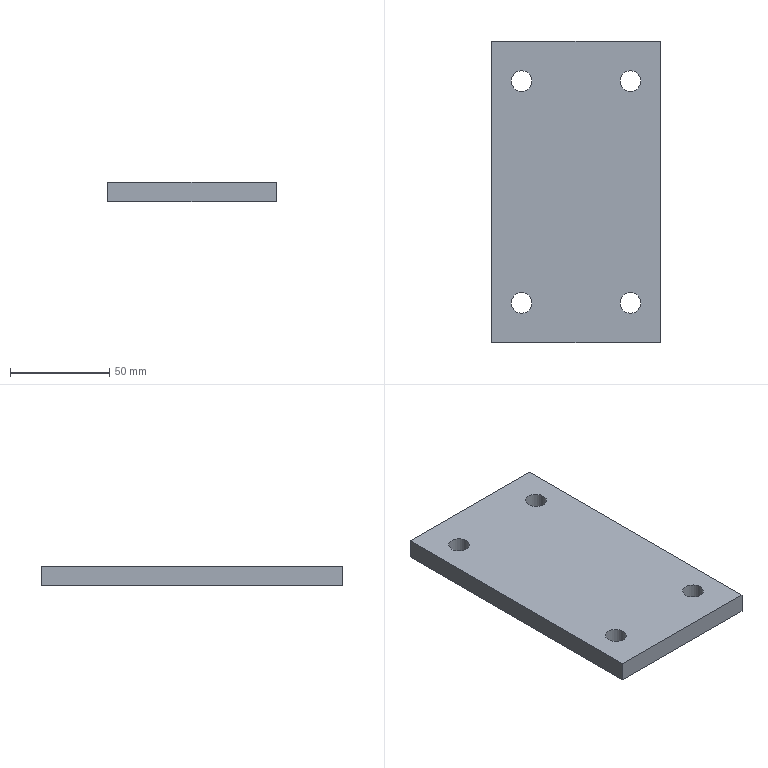Component | NX | FIXED_PLATE_7 | 1 solid | 10 faces | box 85 x 152 x 10 mm | volume 125736 mm3 | plane 6 | cylinder 4 | commonest cylinder face diameters 10.5 x4
STEP:
#1=CARTESIAN_POINT('',(0.,0.,0.));
#2=DIRECTION('',(0.,0.,1.));
#3=DIRECTION('',(1.,0.,0.));
#4=AXIS2_PLACEMENT_3D('',#1,#2,#3);
#5=CARTESIAN_POINT('',(1381.754,1330.,781.574));
#6=VERTEX_POINT('',#5);
#7=CARTESIAN_POINT('',(1381.754,1178.,781.574));
#8=VERTEX_POINT('',#7);
#9=CARTESIAN_POINT('',(1381.754,1330.,781.574));
#10=DIRECTION('',(0.,-1.,0.));
#11=VECTOR('',#10,1.);
#12=LINE('',#9,#11);
#13=CARTESIAN_POINT('',(1381.754,1330.,771.574));
#14=DIRECTION('',(-1.,0.,0.));
#15=DIRECTION('',(0.,0.,1.));
#16=AXIS2_PLACEMENT_3D('',#13,#14,#15);
#17=PLANE('',#16);
#18=CARTESIAN_POINT('',(10.,0.));
#19=DIRECTION('',(0.,-1.));
#20=VECTOR('',#19,1.);
#21=LINE('',#18,#20);
#22=(GEOMETRIC_REPRESENTATION_CONTEXT(2)PARAMETRIC_REPRESENTATION_CONTEXT()REPRESENTATION_CONTEXT('',''));
#23=DEFINITIONAL_REPRESENTATION('',(#21),#22);
#24=PCURVE('',#17,#23);
#25=CARTESIAN_POINT('',(1396.754,1198.,781.574));
#26=DIRECTION('',(0.,0.,1.));
#27=DIRECTION('',(1.,0.,0.));
#28=AXIS2_PLACEMENT_3D('',#25,#26,#27);
#29=PLANE('',#28);
#30=CARTESIAN_POINT('',(-15.,132.));
#31=DIRECTION('',(0.,-1.));
#32=VECTOR('',#31,1.);
#33=LINE('',#30,#32);
#34=(GEOMETRIC_REPRESENTATION_CONTEXT(2)PARAMETRIC_REPRESENTATION_CONTEXT()REPRESENTATION_CONTEXT('',''));
#35=DEFINITIONAL_REPRESENTATION('',(#33),#34);
#36=PCURVE('',#29,#35);
#37=SURFACE_CURVE('',#12,(#24,#36),.PCURVE_S1.);
#38=EDGE_CURVE('',#6,#8,#37,.T.);
#39=ORIENTED_EDGE('',*,*,#38,.F.);
#40=CARTESIAN_POINT('',(1381.754,1330.,771.574));
#41=VERTEX_POINT('',#40);
#42=CARTESIAN_POINT('',(1381.754,1330.,771.574));
#43=DIRECTION('',(0.,0.,1.));
#44=VECTOR('',#43,1.);
#45=LINE('',#42,#44);
#46=CARTESIAN_POINT('',(0.,0.));
#47=DIRECTION('',(1.,0.));
#48=VECTOR('',#47,1.);
#49=LINE('',#46,#48);
#50=(GEOMETRIC_REPRESENTATION_CONTEXT(2)PARAMETRIC_REPRESENTATION_CONTEXT()REPRESENTATION_CONTEXT('',''));
#51=DEFINITIONAL_REPRESENTATION('',(#49),#50);
#52=PCURVE('',#17,#51);
#53=CARTESIAN_POINT('',(1466.754,1330.,771.574));
#54=DIRECTION('',(0.,1.,0.));
#55=DIRECTION('',(0.,0.,1.));
#56=AXIS2_PLACEMENT_3D('',#53,#54,#55);
#57=PLANE('',#56);
#58=CARTESIAN_POINT('',(0.,-85.));
#59=DIRECTION('',(1.,0.));
#60=VECTOR('',#59,1.);
#61=LINE('',#58,#60);
#62=(GEOMETRIC_REPRESENTATION_CONTEXT(2)PARAMETRIC_REPRESENTATION_CONTEXT()REPRESENTATION_CONTEXT('',''));
#63=DEFINITIONAL_REPRESENTATION('',(#61),#62);
#64=PCURVE('',#57,#63);
#65=SURFACE_CURVE('',#45,(#52,#64),.PCURVE_S1.);
#66=EDGE_CURVE('',#41,#6,#65,.T.);
#67=ORIENTED_EDGE('',*,*,#66,.F.);
#68=CARTESIAN_POINT('',(1381.754,1178.,771.574));
#69=VERTEX_POINT('',#68);
#70=CARTESIAN_POINT('',(1381.754,1330.,771.574));
#71=DIRECTION('',(0.,-1.,0.));
#72=VECTOR('',#71,1.);
#73=LINE('',#70,#72);
#74=CARTESIAN_POINT('',(0.,0.));
#75=DIRECTION('',(0.,-1.));
#76=VECTOR('',#75,1.);
#77=LINE('',#74,#76);
#78=(GEOMETRIC_REPRESENTATION_CONTEXT(2)PARAMETRIC_REPRESENTATION_CONTEXT()REPRESENTATION_CONTEXT('',''));
#79=DEFINITIONAL_REPRESENTATION('',(#77),#78);
#80=PCURVE('',#17,#79);
#81=CARTESIAN_POINT('',(1396.754,1198.,771.574));
#82=DIRECTION('',(0.,0.,1.));
#83=DIRECTION('',(1.,0.,0.));
#84=AXIS2_PLACEMENT_3D('',#81,#82,#83);
#85=PLANE('',#84);
#86=CARTESIAN_POINT('',(-15.,132.));
#87=DIRECTION('',(0.,-1.));
#88=VECTOR('',#87,1.);
#89=LINE('',#86,#88);
#90=(GEOMETRIC_REPRESENTATION_CONTEXT(2)PARAMETRIC_REPRESENTATION_CONTEXT()REPRESENTATION_CONTEXT('',''));
#91=DEFINITIONAL_REPRESENTATION('',(#89),#90);
#92=PCURVE('',#85,#91);
#93=SURFACE_CURVE('',#73,(#80,#92),.PCURVE_S1.);
#94=EDGE_CURVE('',#41,#69,#93,.T.);
#95=ORIENTED_EDGE('',*,*,#94,.T.);
#96=CARTESIAN_POINT('',(1381.754,1178.,771.574));
#97=DIRECTION('',(0.,0.,1.));
#98=VECTOR('',#97,1.);
#99=LINE('',#96,#98);
#100=CARTESIAN_POINT('',(0.,-152.));
#101=DIRECTION('',(1.,0.));
#102=VECTOR('',#101,1.);
#103=LINE('',#100,#102);
#104=(GEOMETRIC_REPRESENTATION_CONTEXT(2)PARAMETRIC_REPRESENTATION_CONTEXT()REPRESENTATION_CONTEXT('',''));
#105=DEFINITIONAL_REPRESENTATION('',(#103),#104);
#106=PCURVE('',#17,#105);
#107=CARTESIAN_POINT('',(1381.754,1178.,771.574));
#108=DIRECTION('',(0.,-1.,0.));
#109=DIRECTION('',(0.,0.,-1.));
#110=AXIS2_PLACEMENT_3D('',#107,#108,#109);
#111=PLANE('',#110);
#112=CARTESIAN_POINT('',(0.,0.));
#113=DIRECTION('',(-1.,0.));
#114=VECTOR('',#113,1.);
#115=LINE('',#112,#114);
#116=(GEOMETRIC_REPRESENTATION_CONTEXT(2)PARAMETRIC_REPRESENTATION_CONTEXT()REPRESENTATION_CONTEXT('',''));
#117=DEFINITIONAL_REPRESENTATION('',(#115),#116);
#118=PCURVE('',#111,#117);
#119=SURFACE_CURVE('',#99,(#106,#118),.PCURVE_S1.);
#120=EDGE_CURVE('',#69,#8,#119,.T.);
#121=ORIENTED_EDGE('',*,*,#120,.T.);
#122=EDGE_LOOP('',(#39,#67,#95,#121));
#123=FACE_BOUND('',#122,.T.);
#124=ADVANCED_FACE('',(#123),#17,.T.);
#125=CARTESIAN_POINT('',(1466.754,1178.,781.574));
#126=VERTEX_POINT('',#125);
#127=CARTESIAN_POINT('',(1381.754,1178.,781.574));
#128=DIRECTION('',(1.,0.,0.));
#129=VECTOR('',#128,1.);
#130=LINE('',#127,#129);
#131=CARTESIAN_POINT('',(-10.,0.));
#132=DIRECTION('',(0.,1.));
#133=VECTOR('',#132,1.);
#134=LINE('',#131,#133);
#135=(GEOMETRIC_REPRESENTATION_CONTEXT(2)PARAMETRIC_REPRESENTATION_CONTEXT()REPRESENTATION_CONTEXT('',''));
#136=DEFINITIONAL_REPRESENTATION('',(#134),#135);
#137=PCURVE('',#111,#136);
#138=CARTESIAN_POINT('',(-15.,-20.));
#139=DIRECTION('',(1.,0.));
#140=VECTOR('',#139,1.);
#141=LINE('',#138,#140);
#142=(GEOMETRIC_REPRESENTATION_CONTEXT(2)PARAMETRIC_REPRESENTATION_CONTEXT()REPRESENTATION_CONTEXT('',''));
#143=DEFINITIONAL_REPRESENTATION('',(#141),#142);
#144=PCURVE('',#29,#143);
#145=SURFACE_CURVE('',#130,(#137,#144),.PCURVE_S1.);
#146=EDGE_CURVE('',#8,#126,#145,.T.);
#147=ORIENTED_EDGE('',*,*,#146,.F.);
#148=ORIENTED_EDGE('',*,*,#120,.F.);
#149=CARTESIAN_POINT('',(1466.754,1178.,771.574));
#150=VERTEX_POINT('',#149);
#151=CARTESIAN_POINT('',(1381.754,1178.,771.574));
#152=DIRECTION('',(1.,0.,0.));
#153=VECTOR('',#152,1.);
#154=LINE('',#151,#153);
#155=CARTESIAN_POINT('',(0.,0.));
#156=DIRECTION('',(0.,1.));
#157=VECTOR('',#156,1.);
#158=LINE('',#155,#157);
#159=(GEOMETRIC_REPRESENTATION_CONTEXT(2)PARAMETRIC_REPRESENTATION_CONTEXT()REPRESENTATION_CONTEXT('',''));
#160=DEFINITIONAL_REPRESENTATION('',(#158),#159);
#161=PCURVE('',#111,#160);
#162=CARTESIAN_POINT('',(-15.,-20.));
#163=DIRECTION('',(1.,0.));
#164=VECTOR('',#163,1.);
#165=LINE('',#162,#164);
#166=(GEOMETRIC_REPRESENTATION_CONTEXT(2)PARAMETRIC_REPRESENTATION_CONTEXT()REPRESENTATION_CONTEXT('',''));
#167=DEFINITIONAL_REPRESENTATION('',(#165),#166);
#168=PCURVE('',#85,#167);
#169=SURFACE_CURVE('',#154,(#161,#168),.PCURVE_S1.);
#170=EDGE_CURVE('',#69,#150,#169,.T.);
#171=ORIENTED_EDGE('',*,*,#170,.T.);
#172=CARTESIAN_POINT('',(1466.754,1178.,771.574));
#173=DIRECTION('',(0.,0.,1.));
#174=VECTOR('',#173,1.);
#175=LINE('',#172,#174);
#176=CARTESIAN_POINT('',(0.,85.));
#177=DIRECTION('',(-1.,0.));
#178=VECTOR('',#177,1.);
#179=LINE('',#176,#178);
#180=(GEOMETRIC_REPRESENTATION_CONTEXT(2)PARAMETRIC_REPRESENTATION_CONTEXT()REPRESENTATION_CONTEXT('',''));
#181=DEFINITIONAL_REPRESENTATION('',(#179),#180);
#182=PCURVE('',#111,#181);
#183=CARTESIAN_POINT('',(1466.754,1178.,771.574));
#184=DIRECTION('',(1.,-0.,0.));
#185=DIRECTION('',(0.,1.,0.));
#186=AXIS2_PLACEMENT_3D('',#183,#184,#185);
#187=PLANE('',#186);
#188=CARTESIAN_POINT('',(0.,0.));
#189=DIRECTION('',(0.,1.));
#190=VECTOR('',#189,1.);
#191=LINE('',#188,#190);
#192=(GEOMETRIC_REPRESENTATION_CONTEXT(2)PARAMETRIC_REPRESENTATION_CONTEXT()REPRESENTATION_CONTEXT('',''));
#193=DEFINITIONAL_REPRESENTATION('',(#191),#192);
#194=PCURVE('',#187,#193);
#195=SURFACE_CURVE('',#175,(#182,#194),.PCURVE_S1.);
#196=EDGE_CURVE('',#150,#126,#195,.T.);
#197=ORIENTED_EDGE('',*,*,#196,.T.);
#198=EDGE_LOOP('',(#147,#148,#171,#197));
#199=FACE_BOUND('',#198,.T.);
#200=ADVANCED_FACE('',(#199),#111,.T.);
#201=CARTESIAN_POINT('',(1466.754,1330.,781.574));
#202=VERTEX_POINT('',#201);
#203=CARTESIAN_POINT('',(1466.754,1178.,781.574));
#204=DIRECTION('',(0.,1.,0.));
#205=VECTOR('',#204,1.);
#206=LINE('',#203,#205);
#207=CARTESIAN_POINT('',(0.,10.));
#208=DIRECTION('',(1.,0.));
#209=VECTOR('',#208,1.);
#210=LINE('',#207,#209);
#211=(GEOMETRIC_REPRESENTATION_CONTEXT(2)PARAMETRIC_REPRESENTATION_CONTEXT()REPRESENTATION_CONTEXT('',''));
#212=DEFINITIONAL_REPRESENTATION('',(#210),#211);
#213=PCURVE('',#187,#212);
#214=CARTESIAN_POINT('',(70.,-20.));
#215=DIRECTION('',(0.,1.));
#216=VECTOR('',#215,1.);
#217=LINE('',#214,#216);
#218=(GEOMETRIC_REPRESENTATION_CONTEXT(2)PARAMETRIC_REPRESENTATION_CONTEXT()REPRESENTATION_CONTEXT('',''));
#219=DEFINITIONAL_REPRESENTATION('',(#217),#218);
#220=PCURVE('',#29,#219);
#221=SURFACE_CURVE('',#206,(#213,#220),.PCURVE_S1.);
#222=EDGE_CURVE('',#126,#202,#221,.T.);
#223=ORIENTED_EDGE('',*,*,#222,.F.);
#224=ORIENTED_EDGE('',*,*,#196,.F.);
#225=CARTESIAN_POINT('',(1466.754,1330.,771.574));
#226=VERTEX_POINT('',#225);
#227=CARTESIAN_POINT('',(1466.754,1178.,771.574));
#228=DIRECTION('',(0.,1.,0.));
#229=VECTOR('',#228,1.);
#230=LINE('',#227,#229);
#231=CARTESIAN_POINT('',(0.,0.));
#232=DIRECTION('',(1.,0.));
#233=VECTOR('',#232,1.);
#234=LINE('',#231,#233);
#235=(GEOMETRIC_REPRESENTATION_CONTEXT(2)PARAMETRIC_REPRESENTATION_CONTEXT()REPRESENTATION_CONTEXT('',''));
#236=DEFINITIONAL_REPRESENTATION('',(#234),#235);
#237=PCURVE('',#187,#236);
#238=CARTESIAN_POINT('',(70.,-20.));
#239=DIRECTION('',(0.,1.));
#240=VECTOR('',#239,1.);
#241=LINE('',#238,#240);
#242=(GEOMETRIC_REPRESENTATION_CONTEXT(2)PARAMETRIC_REPRESENTATION_CONTEXT()REPRESENTATION_CONTEXT('',''));
#243=DEFINITIONAL_REPRESENTATION('',(#241),#242);
#244=PCURVE('',#85,#243);
#245=SURFACE_CURVE('',#230,(#237,#244),.PCURVE_S1.);
#246=EDGE_CURVE('',#150,#226,#245,.T.);
#247=ORIENTED_EDGE('',*,*,#246,.T.);
#248=CARTESIAN_POINT('',(1466.754,1330.,771.574));
#249=DIRECTION('',(0.,0.,1.));
#250=VECTOR('',#249,1.);
#251=LINE('',#248,#250);
#252=CARTESIAN_POINT('',(152.,0.));
#253=DIRECTION('',(0.,1.));
#254=VECTOR('',#253,1.);
#255=LINE('',#252,#254);
#256=(GEOMETRIC_REPRESENTATION_CONTEXT(2)PARAMETRIC_REPRESENTATION_CONTEXT()REPRESENTATION_CONTEXT('',''));
#257=DEFINITIONAL_REPRESENTATION('',(#255),#256);
#258=PCURVE('',#187,#257);
#259=CARTESIAN_POINT('',(0.,0.));
#260=DIRECTION('',(1.,0.));
#261=VECTOR('',#260,1.);
#262=LINE('',#259,#261);
#263=(GEOMETRIC_REPRESENTATION_CONTEXT(2)PARAMETRIC_REPRESENTATION_CONTEXT()REPRESENTATION_CONTEXT('',''));
#264=DEFINITIONAL_REPRESENTATION('',(#262),#263);
#265=PCURVE('',#57,#264);
#266=SURFACE_CURVE('',#251,(#258,#265),.PCURVE_S1.);
#267=EDGE_CURVE('',#226,#202,#266,.T.);
#268=ORIENTED_EDGE('',*,*,#267,.T.);
#269=EDGE_LOOP('',(#223,#224,#247,#268));
#270=FACE_BOUND('',#269,.T.);
#271=ADVANCED_FACE('',(#270),#187,.T.);
#272=CARTESIAN_POINT('',(1457.004,1198.,771.574));
#273=VERTEX_POINT('',#272);
#274=CARTESIAN_POINT('',(1451.754,1198.,771.574));
#275=DIRECTION('',(0.,0.,1.));
#276=DIRECTION('',(1.,0.,0.));
#277=AXIS2_PLACEMENT_3D('',#274,#275,#276);
#278=CIRCLE('',#277,5.25);
#279=CARTESIAN_POINT('',(1451.754,1198.,771.574));
#280=DIRECTION('',(0.,0.,1.));
#281=DIRECTION('',(1.,0.,0.));
#282=AXIS2_PLACEMENT_3D('',#279,#280,#281);
#283=CYLINDRICAL_SURFACE('',#282,5.25);
#284=CARTESIAN_POINT('',(0.,0.));
#285=DIRECTION('',(1.,0.));
#286=VECTOR('',#285,1.);
#287=LINE('',#284,#286);
#288=(GEOMETRIC_REPRESENTATION_CONTEXT(2)PARAMETRIC_REPRESENTATION_CONTEXT()REPRESENTATION_CONTEXT('',''));
#289=DEFINITIONAL_REPRESENTATION('',(#287),#288);
#290=PCURVE('',#283,#289);
#291=CARTESIAN_POINT('',(55.,0.));
#292=DIRECTION('',(1.,0.));
#293=AXIS2_PLACEMENT_2D('',#291,#292);
#294=CIRCLE('',#293,5.25);
#295=(GEOMETRIC_REPRESENTATION_CONTEXT(2)PARAMETRIC_REPRESENTATION_CONTEXT()REPRESENTATION_CONTEXT('',''));
#296=DEFINITIONAL_REPRESENTATION('',(#294),#295);
#297=PCURVE('',#85,#296);
#298=SURFACE_CURVE('',#278,(#290,#297),.PCURVE_S1.);
#299=EDGE_CURVE('',#273,#273,#298,.T.);
#300=ORIENTED_EDGE('',*,*,#299,.T.);
#301=CARTESIAN_POINT('',(1457.004,1198.,781.574));
#302=VERTEX_POINT('',#301);
#303=CARTESIAN_POINT('',(1457.004,1198.,771.574));
#304=CARTESIAN_POINT('',(1457.004,1198.,781.574));
#305=B_SPLINE_CURVE_WITH_KNOTS('',1,(#303,#304),.UNSPECIFIED.,.F.,.F.,(2,2),(0.,10.),.PIECEWISE_BEZIER_KNOTS.);
#306=CARTESIAN_POINT('',(6.283,0.));
#307=DIRECTION('',(0.,1.));
#308=VECTOR('',#307,1.);
#309=LINE('',#306,#308);
#310=(GEOMETRIC_REPRESENTATION_CONTEXT(2)PARAMETRIC_REPRESENTATION_CONTEXT()REPRESENTATION_CONTEXT('',''));
#311=DEFINITIONAL_REPRESENTATION('',(#309),#310);
#312=PCURVE('',#283,#311);
#313=CARTESIAN_POINT('',(0.,0.));
#314=DIRECTION('',(0.,1.));
#315=VECTOR('',#314,1.);
#316=LINE('',#313,#315);
#317=(GEOMETRIC_REPRESENTATION_CONTEXT(2)PARAMETRIC_REPRESENTATION_CONTEXT()REPRESENTATION_CONTEXT('',''));
#318=DEFINITIONAL_REPRESENTATION('',(#316),#317);
#319=PCURVE('',#283,#318);
#320=SEAM_CURVE('',#305,(#312,#319),.PCURVE_S1.);
#321=EDGE_CURVE('',#273,#302,#320,.T.);
#322=ORIENTED_EDGE('',*,*,#321,.T.);
#323=CARTESIAN_POINT('',(1451.754,1198.,781.574));
#324=DIRECTION('',(0.,0.,1.));
#325=DIRECTION('',(1.,0.,0.));
#326=AXIS2_PLACEMENT_3D('',#323,#324,#325);
#327=CIRCLE('',#326,5.25);
#328=CARTESIAN_POINT('',(0.,10.));
#329=DIRECTION('',(1.,0.));
#330=VECTOR('',#329,1.);
#331=LINE('',#328,#330);
#332=(GEOMETRIC_REPRESENTATION_CONTEXT(2)PARAMETRIC_REPRESENTATION_CONTEXT()REPRESENTATION_CONTEXT('',''));
#333=DEFINITIONAL_REPRESENTATION('',(#331),#332);
#334=PCURVE('',#283,#333);
#335=CARTESIAN_POINT('',(55.,0.));
#336=DIRECTION('',(1.,0.));
#337=AXIS2_PLACEMENT_2D('',#335,#336);
#338=CIRCLE('',#337,5.25);
#339=(GEOMETRIC_REPRESENTATION_CONTEXT(2)PARAMETRIC_REPRESENTATION_CONTEXT()REPRESENTATION_CONTEXT('',''));
#340=DEFINITIONAL_REPRESENTATION('',(#338),#339);
#341=PCURVE('',#29,#340);
#342=SURFACE_CURVE('',#327,(#334,#341),.PCURVE_S1.);
#343=EDGE_CURVE('',#302,#302,#342,.T.);
#344=ORIENTED_EDGE('',*,*,#343,.F.);
#345=ORIENTED_EDGE('',*,*,#321,.F.);
#346=EDGE_LOOP('',(#300,#322,#344,#345));
#347=FACE_BOUND('',#346,.F.);
#348=ADVANCED_FACE('',(#347),#283,.F.);
#349=CARTESIAN_POINT('',(1402.004,1310.,771.574));
#350=VERTEX_POINT('',#349);
#351=CARTESIAN_POINT('',(1396.754,1310.,771.574));
#352=DIRECTION('',(0.,0.,1.));
#353=DIRECTION('',(1.,0.,0.));
#354=AXIS2_PLACEMENT_3D('',#351,#352,#353);
#355=CIRCLE('',#354,5.25);
#356=CARTESIAN_POINT('',(1396.754,1310.,771.574));
#357=DIRECTION('',(0.,0.,1.));
#358=DIRECTION('',(1.,0.,0.));
#359=AXIS2_PLACEMENT_3D('',#356,#357,#358);
#360=CYLINDRICAL_SURFACE('',#359,5.25);
#361=CARTESIAN_POINT('',(0.,0.));
#362=DIRECTION('',(1.,0.));
#363=VECTOR('',#362,1.);
#364=LINE('',#361,#363);
#365=(GEOMETRIC_REPRESENTATION_CONTEXT(2)PARAMETRIC_REPRESENTATION_CONTEXT()REPRESENTATION_CONTEXT('',''));
#366=DEFINITIONAL_REPRESENTATION('',(#364),#365);
#367=PCURVE('',#360,#366);
#368=CARTESIAN_POINT('',(0.,112.));
#369=DIRECTION('',(1.,0.));
#370=AXIS2_PLACEMENT_2D('',#368,#369);
#371=CIRCLE('',#370,5.25);
#372=(GEOMETRIC_REPRESENTATION_CONTEXT(2)PARAMETRIC_REPRESENTATION_CONTEXT()REPRESENTATION_CONTEXT('',''));
#373=DEFINITIONAL_REPRESENTATION('',(#371),#372);
#374=PCURVE('',#85,#373);
#375=SURFACE_CURVE('',#355,(#367,#374),.PCURVE_S1.);
#376=EDGE_CURVE('',#350,#350,#375,.T.);
#377=ORIENTED_EDGE('',*,*,#376,.T.);
#378=CARTESIAN_POINT('',(1402.004,1310.,781.574));
#379=VERTEX_POINT('',#378);
#380=CARTESIAN_POINT('',(1402.004,1310.,771.574));
#381=CARTESIAN_POINT('',(1402.004,1310.,781.574));
#382=B_SPLINE_CURVE_WITH_KNOTS('',1,(#380,#381),.UNSPECIFIED.,.F.,.F.,(2,2),(0.,10.),.PIECEWISE_BEZIER_KNOTS.);
#383=CARTESIAN_POINT('',(6.283,0.));
#384=DIRECTION('',(0.,1.));
#385=VECTOR('',#384,1.);
#386=LINE('',#383,#385);
#387=(GEOMETRIC_REPRESENTATION_CONTEXT(2)PARAMETRIC_REPRESENTATION_CONTEXT()REPRESENTATION_CONTEXT('',''));
#388=DEFINITIONAL_REPRESENTATION('',(#386),#387);
#389=PCURVE('',#360,#388);
#390=CARTESIAN_POINT('',(0.,0.));
#391=DIRECTION('',(0.,1.));
#392=VECTOR('',#391,1.);
#393=LINE('',#390,#392);
#394=(GEOMETRIC_REPRESENTATION_CONTEXT(2)PARAMETRIC_REPRESENTATION_CONTEXT()REPRESENTATION_CONTEXT('',''));
#395=DEFINITIONAL_REPRESENTATION('',(#393),#394);
#396=PCURVE('',#360,#395);
#397=SEAM_CURVE('',#382,(#389,#396),.PCURVE_S1.);
#398=EDGE_CURVE('',#350,#379,#397,.T.);
#399=ORIENTED_EDGE('',*,*,#398,.T.);
#400=CARTESIAN_POINT('',(1396.754,1310.,781.574));
#401=DIRECTION('',(0.,0.,1.));
#402=DIRECTION('',(1.,0.,0.));
#403=AXIS2_PLACEMENT_3D('',#400,#401,#402);
#404=CIRCLE('',#403,5.25);
#405=CARTESIAN_POINT('',(0.,10.));
#406=DIRECTION('',(1.,0.));
#407=VECTOR('',#406,1.);
#408=LINE('',#405,#407);
#409=(GEOMETRIC_REPRESENTATION_CONTEXT(2)PARAMETRIC_REPRESENTATION_CONTEXT()REPRESENTATION_CONTEXT('',''));
#410=DEFINITIONAL_REPRESENTATION('',(#408),#409);
#411=PCURVE('',#360,#410);
#412=CARTESIAN_POINT('',(0.,112.));
#413=DIRECTION('',(1.,0.));
#414=AXIS2_PLACEMENT_2D('',#412,#413);
#415=CIRCLE('',#414,5.25);
#416=(GEOMETRIC_REPRESENTATION_CONTEXT(2)PARAMETRIC_REPRESENTATION_CONTEXT()REPRESENTATION_CONTEXT('',''));
#417=DEFINITIONAL_REPRESENTATION('',(#415),#416);
#418=PCURVE('',#29,#417);
#419=SURFACE_CURVE('',#404,(#411,#418),.PCURVE_S1.);
#420=EDGE_CURVE('',#379,#379,#419,.T.);
#421=ORIENTED_EDGE('',*,*,#420,.F.);
#422=ORIENTED_EDGE('',*,*,#398,.F.);
#423=EDGE_LOOP('',(#377,#399,#421,#422));
#424=FACE_BOUND('',#423,.F.);
#425=ADVANCED_FACE('',(#424),#360,.F.);
#426=CARTESIAN_POINT('',(1402.004,1198.,771.574));
#427=VERTEX_POINT('',#426);
#428=CARTESIAN_POINT('',(1396.754,1198.,771.574));
#429=DIRECTION('',(0.,0.,1.));
#430=DIRECTION('',(1.,0.,0.));
#431=AXIS2_PLACEMENT_3D('',#428,#429,#430);
#432=CIRCLE('',#431,5.25);
#433=CARTESIAN_POINT('',(1396.754,1198.,771.574));
#434=DIRECTION('',(0.,0.,1.));
#435=DIRECTION('',(1.,0.,0.));
#436=AXIS2_PLACEMENT_3D('',#433,#434,#435);
#437=CYLINDRICAL_SURFACE('',#436,5.25);
#438=CARTESIAN_POINT('',(0.,0.));
#439=DIRECTION('',(1.,0.));
#440=VECTOR('',#439,1.);
#441=LINE('',#438,#440);
#442=(GEOMETRIC_REPRESENTATION_CONTEXT(2)PARAMETRIC_REPRESENTATION_CONTEXT()REPRESENTATION_CONTEXT('',''));
#443=DEFINITIONAL_REPRESENTATION('',(#441),#442);
#444=PCURVE('',#437,#443);
#445=CARTESIAN_POINT('',(0.,0.));
#446=DIRECTION('',(1.,0.));
#447=AXIS2_PLACEMENT_2D('',#445,#446);
#448=CIRCLE('',#447,5.25);
#449=(GEOMETRIC_REPRESENTATION_CONTEXT(2)PARAMETRIC_REPRESENTATION_CONTEXT()REPRESENTATION_CONTEXT('',''));
#450=DEFINITIONAL_REPRESENTATION('',(#448),#449);
#451=PCURVE('',#85,#450);
#452=SURFACE_CURVE('',#432,(#444,#451),.PCURVE_S1.);
#453=EDGE_CURVE('',#427,#427,#452,.T.);
#454=ORIENTED_EDGE('',*,*,#453,.T.);
#455=CARTESIAN_POINT('',(1402.004,1198.,781.574));
#456=VERTEX_POINT('',#455);
#457=CARTESIAN_POINT('',(1402.004,1198.,771.574));
#458=CARTESIAN_POINT('',(1402.004,1198.,781.574));
#459=B_SPLINE_CURVE_WITH_KNOTS('',1,(#457,#458),.UNSPECIFIED.,.F.,.F.,(2,2),(0.,10.),.PIECEWISE_BEZIER_KNOTS.);
#460=CARTESIAN_POINT('',(6.283,0.));
#461=DIRECTION('',(0.,1.));
#462=VECTOR('',#461,1.);
#463=LINE('',#460,#462);
#464=(GEOMETRIC_REPRESENTATION_CONTEXT(2)PARAMETRIC_REPRESENTATION_CONTEXT()REPRESENTATION_CONTEXT('',''));
#465=DEFINITIONAL_REPRESENTATION('',(#463),#464);
#466=PCURVE('',#437,#465);
#467=CARTESIAN_POINT('',(0.,0.));
#468=DIRECTION('',(0.,1.));
#469=VECTOR('',#468,1.);
#470=LINE('',#467,#469);
#471=(GEOMETRIC_REPRESENTATION_CONTEXT(2)PARAMETRIC_REPRESENTATION_CONTEXT()REPRESENTATION_CONTEXT('',''));
#472=DEFINITIONAL_REPRESENTATION('',(#470),#471);
#473=PCURVE('',#437,#472);
#474=SEAM_CURVE('',#459,(#466,#473),.PCURVE_S1.);
#475=EDGE_CURVE('',#427,#456,#474,.T.);
#476=ORIENTED_EDGE('',*,*,#475,.T.);
#477=CARTESIAN_POINT('',(1396.754,1198.,781.574));
#478=DIRECTION('',(0.,0.,1.));
#479=DIRECTION('',(1.,0.,0.));
#480=AXIS2_PLACEMENT_3D('',#477,#478,#479);
#481=CIRCLE('',#480,5.25);
#482=CARTESIAN_POINT('',(0.,10.));
#483=DIRECTION('',(1.,0.));
#484=VECTOR('',#483,1.);
#485=LINE('',#482,#484);
#486=(GEOMETRIC_REPRESENTATION_CONTEXT(2)PARAMETRIC_REPRESENTATION_CONTEXT()REPRESENTATION_CONTEXT('',''));
#487=DEFINITIONAL_REPRESENTATION('',(#485),#486);
#488=PCURVE('',#437,#487);
#489=CARTESIAN_POINT('',(0.,0.));
#490=DIRECTION('',(1.,0.));
#491=AXIS2_PLACEMENT_2D('',#489,#490);
#492=CIRCLE('',#491,5.25);
#493=(GEOMETRIC_REPRESENTATION_CONTEXT(2)PARAMETRIC_REPRESENTATION_CONTEXT()REPRESENTATION_CONTEXT('',''));
#494=DEFINITIONAL_REPRESENTATION('',(#492),#493);
#495=PCURVE('',#29,#494);
#496=SURFACE_CURVE('',#481,(#488,#495),.PCURVE_S1.);
#497=EDGE_CURVE('',#456,#456,#496,.T.);
#498=ORIENTED_EDGE('',*,*,#497,.F.);
#499=ORIENTED_EDGE('',*,*,#475,.F.);
#500=EDGE_LOOP('',(#454,#476,#498,#499));
#501=FACE_BOUND('',#500,.F.);
#502=ADVANCED_FACE('',(#501),#437,.F.);
#503=CARTESIAN_POINT('',(1466.754,1330.,781.574));
#504=DIRECTION('',(-1.,0.,0.));
#505=VECTOR('',#504,1.);
#506=LINE('',#503,#505);
#507=CARTESIAN_POINT('',(10.,0.));
#508=DIRECTION('',(0.,-1.));
#509=VECTOR('',#508,1.);
#510=LINE('',#507,#509);
#511=(GEOMETRIC_REPRESENTATION_CONTEXT(2)PARAMETRIC_REPRESENTATION_CONTEXT()REPRESENTATION_CONTEXT('',''));
#512=DEFINITIONAL_REPRESENTATION('',(#510),#511);
#513=PCURVE('',#57,#512);
#514=CARTESIAN_POINT('',(70.,132.));
#515=DIRECTION('',(-1.,0.));
#516=VECTOR('',#515,1.);
#517=LINE('',#514,#516);
#518=(GEOMETRIC_REPRESENTATION_CONTEXT(2)PARAMETRIC_REPRESENTATION_CONTEXT()REPRESENTATION_CONTEXT('',''));
#519=DEFINITIONAL_REPRESENTATION('',(#517),#518);
#520=PCURVE('',#29,#519);
#521=SURFACE_CURVE('',#506,(#513,#520),.PCURVE_S1.);
#522=EDGE_CURVE('',#202,#6,#521,.T.);
#523=ORIENTED_EDGE('',*,*,#522,.F.);
#524=ORIENTED_EDGE('',*,*,#267,.F.);
#525=CARTESIAN_POINT('',(1466.754,1330.,771.574));
#526=DIRECTION('',(-1.,0.,0.));
#527=VECTOR('',#526,1.);
#528=LINE('',#525,#527);
#529=CARTESIAN_POINT('',(0.,0.));
#530=DIRECTION('',(0.,-1.));
#531=VECTOR('',#530,1.);
#532=LINE('',#529,#531);
#533=(GEOMETRIC_REPRESENTATION_CONTEXT(2)PARAMETRIC_REPRESENTATION_CONTEXT()REPRESENTATION_CONTEXT('',''));
#534=DEFINITIONAL_REPRESENTATION('',(#532),#533);
#535=PCURVE('',#57,#534);
#536=CARTESIAN_POINT('',(70.,132.));
#537=DIRECTION('',(-1.,0.));
#538=VECTOR('',#537,1.);
#539=LINE('',#536,#538);
#540=(GEOMETRIC_REPRESENTATION_CONTEXT(2)PARAMETRIC_REPRESENTATION_CONTEXT()REPRESENTATION_CONTEXT('',''));
#541=DEFINITIONAL_REPRESENTATION('',(#539),#540);
#542=PCURVE('',#85,#541);
#543=SURFACE_CURVE('',#528,(#535,#542),.PCURVE_S1.);
#544=EDGE_CURVE('',#226,#41,#543,.T.);
#545=ORIENTED_EDGE('',*,*,#544,.T.);
#546=ORIENTED_EDGE('',*,*,#66,.T.);
#547=EDGE_LOOP('',(#523,#524,#545,#546));
#548=FACE_BOUND('',#547,.T.);
#549=ADVANCED_FACE('',(#548),#57,.T.);
#550=CARTESIAN_POINT('',(1457.004,1310.,771.574));
#551=VERTEX_POINT('',#550);
#552=CARTESIAN_POINT('',(1451.754,1310.,771.574));
#553=DIRECTION('',(0.,0.,1.));
#554=DIRECTION('',(1.,0.,0.));
#555=AXIS2_PLACEMENT_3D('',#552,#553,#554);
#556=CIRCLE('',#555,5.25);
#557=CARTESIAN_POINT('',(1451.754,1310.,771.574));
#558=DIRECTION('',(0.,0.,1.));
#559=DIRECTION('',(1.,0.,0.));
#560=AXIS2_PLACEMENT_3D('',#557,#558,#559);
#561=CYLINDRICAL_SURFACE('',#560,5.25);
#562=CARTESIAN_POINT('',(0.,0.));
#563=DIRECTION('',(1.,0.));
#564=VECTOR('',#563,1.);
#565=LINE('',#562,#564);
#566=(GEOMETRIC_REPRESENTATION_CONTEXT(2)PARAMETRIC_REPRESENTATION_CONTEXT()REPRESENTATION_CONTEXT('',''));
#567=DEFINITIONAL_REPRESENTATION('',(#565),#566);
#568=PCURVE('',#561,#567);
#569=CARTESIAN_POINT('',(55.,112.));
#570=DIRECTION('',(1.,0.));
#571=AXIS2_PLACEMENT_2D('',#569,#570);
#572=CIRCLE('',#571,5.25);
#573=(GEOMETRIC_REPRESENTATION_CONTEXT(2)PARAMETRIC_REPRESENTATION_CONTEXT()REPRESENTATION_CONTEXT('',''));
#574=DEFINITIONAL_REPRESENTATION('',(#572),#573);
#575=PCURVE('',#85,#574);
#576=SURFACE_CURVE('',#556,(#568,#575),.PCURVE_S1.);
#577=EDGE_CURVE('',#551,#551,#576,.T.);
#578=ORIENTED_EDGE('',*,*,#577,.T.);
#579=CARTESIAN_POINT('',(1457.004,1310.,781.574));
#580=VERTEX_POINT('',#579);
#581=CARTESIAN_POINT('',(1457.004,1310.,771.574));
#582=CARTESIAN_POINT('',(1457.004,1310.,781.574));
#583=B_SPLINE_CURVE_WITH_KNOTS('',1,(#581,#582),.UNSPECIFIED.,.F.,.F.,(2,2),(0.,10.),.PIECEWISE_BEZIER_KNOTS.);
#584=CARTESIAN_POINT('',(6.283,0.));
#585=DIRECTION('',(0.,1.));
#586=VECTOR('',#585,1.);
#587=LINE('',#584,#586);
#588=(GEOMETRIC_REPRESENTATION_CONTEXT(2)PARAMETRIC_REPRESENTATION_CONTEXT()REPRESENTATION_CONTEXT('',''));
#589=DEFINITIONAL_REPRESENTATION('',(#587),#588);
#590=PCURVE('',#561,#589);
#591=CARTESIAN_POINT('',(0.,0.));
#592=DIRECTION('',(0.,1.));
#593=VECTOR('',#592,1.);
#594=LINE('',#591,#593);
#595=(GEOMETRIC_REPRESENTATION_CONTEXT(2)PARAMETRIC_REPRESENTATION_CONTEXT()REPRESENTATION_CONTEXT('',''));
#596=DEFINITIONAL_REPRESENTATION('',(#594),#595);
#597=PCURVE('',#561,#596);
#598=SEAM_CURVE('',#583,(#590,#597),.PCURVE_S1.);
#599=EDGE_CURVE('',#551,#580,#598,.T.);
#600=ORIENTED_EDGE('',*,*,#599,.T.);
#601=CARTESIAN_POINT('',(1451.754,1310.,781.574));
#602=DIRECTION('',(0.,0.,1.));
#603=DIRECTION('',(1.,0.,0.));
#604=AXIS2_PLACEMENT_3D('',#601,#602,#603);
#605=CIRCLE('',#604,5.25);
#606=CARTESIAN_POINT('',(0.,10.));
#607=DIRECTION('',(1.,0.));
#608=VECTOR('',#607,1.);
#609=LINE('',#606,#608);
#610=(GEOMETRIC_REPRESENTATION_CONTEXT(2)PARAMETRIC_REPRESENTATION_CONTEXT()REPRESENTATION_CONTEXT('',''));
#611=DEFINITIONAL_REPRESENTATION('',(#609),#610);
#612=PCURVE('',#561,#611);
#613=CARTESIAN_POINT('',(55.,112.));
#614=DIRECTION('',(1.,0.));
#615=AXIS2_PLACEMENT_2D('',#613,#614);
#616=CIRCLE('',#615,5.25);
#617=(GEOMETRIC_REPRESENTATION_CONTEXT(2)PARAMETRIC_REPRESENTATION_CONTEXT()REPRESENTATION_CONTEXT('',''));
#618=DEFINITIONAL_REPRESENTATION('',(#616),#617);
#619=PCURVE('',#29,#618);
#620=SURFACE_CURVE('',#605,(#612,#619),.PCURVE_S1.);
#621=EDGE_CURVE('',#580,#580,#620,.T.);
#622=ORIENTED_EDGE('',*,*,#621,.F.);
#623=ORIENTED_EDGE('',*,*,#599,.F.);
#624=EDGE_LOOP('',(#578,#600,#622,#623));
#625=FACE_BOUND('',#624,.F.);
#626=ADVANCED_FACE('',(#625),#561,.F.);
#627=ORIENTED_EDGE('',*,*,#94,.F.);
#628=ORIENTED_EDGE('',*,*,#544,.F.);
#629=ORIENTED_EDGE('',*,*,#246,.F.);
#630=ORIENTED_EDGE('',*,*,#170,.F.);
#631=EDGE_LOOP('',(#627,#628,#629,#630));
#632=FACE_BOUND('',#631,.T.);
#633=ORIENTED_EDGE('',*,*,#453,.T.);
#634=EDGE_LOOP('',(#633));
#635=FACE_BOUND('',#634,.T.);
#636=ORIENTED_EDGE('',*,*,#376,.T.);
#637=EDGE_LOOP('',(#636));
#638=FACE_BOUND('',#637,.T.);
#639=ORIENTED_EDGE('',*,*,#299,.T.);
#640=EDGE_LOOP('',(#639));
#641=FACE_BOUND('',#640,.T.);
#642=ORIENTED_EDGE('',*,*,#577,.T.);
#643=EDGE_LOOP('',(#642));
#644=FACE_BOUND('',#643,.T.);
#645=ADVANCED_FACE('',(#632,#635,#638,#641,#644),#85,.F.);
#646=ORIENTED_EDGE('',*,*,#38,.T.);
#647=ORIENTED_EDGE('',*,*,#146,.T.);
#648=ORIENTED_EDGE('',*,*,#222,.T.);
#649=ORIENTED_EDGE('',*,*,#522,.T.);
#650=EDGE_LOOP('',(#646,#647,#648,#649));
#651=FACE_BOUND('',#650,.T.);
#652=ORIENTED_EDGE('',*,*,#497,.F.);
#653=EDGE_LOOP('',(#652));
#654=FACE_BOUND('',#653,.T.);
#655=ORIENTED_EDGE('',*,*,#420,.F.);
#656=EDGE_LOOP('',(#655));
#657=FACE_BOUND('',#656,.T.);
#658=ORIENTED_EDGE('',*,*,#343,.F.);
#659=EDGE_LOOP('',(#658));
#660=FACE_BOUND('',#659,.T.);
#661=ORIENTED_EDGE('',*,*,#621,.F.);
#662=EDGE_LOOP('',(#661));
#663=FACE_BOUND('',#662,.T.);
#664=ADVANCED_FACE('',(#651,#654,#657,#660,#663),#29,.T.);
#665=CLOSED_SHELL('',(#124,#200,#271,#348,#425,#502,#549,#626,#645,#664));
#666=MANIFOLD_SOLID_BREP('',#665);
#667=(LENGTH_UNIT()NAMED_UNIT(*)SI_UNIT(.MILLI.,.METRE.));
#668=UNCERTAINTY_MEASURE_WITH_UNIT(LENGTH_MEASURE(0.000005),#667,'','');
#669=(NAMED_UNIT(*)PLANE_ANGLE_UNIT()SI_UNIT($,.RADIAN.));
#670=(NAMED_UNIT(*)SI_UNIT($,.STERADIAN.)SOLID_ANGLE_UNIT());
#671=(GEOMETRIC_REPRESENTATION_CONTEXT(3)GLOBAL_UNCERTAINTY_ASSIGNED_CONTEXT((#668))GLOBAL_UNIT_ASSIGNED_CONTEXT((#667,#669,#670))REPRESENTATION_CONTEXT('',''));
#672=ADVANCED_BREP_SHAPE_REPRESENTATION('',(#4,#666),#671);